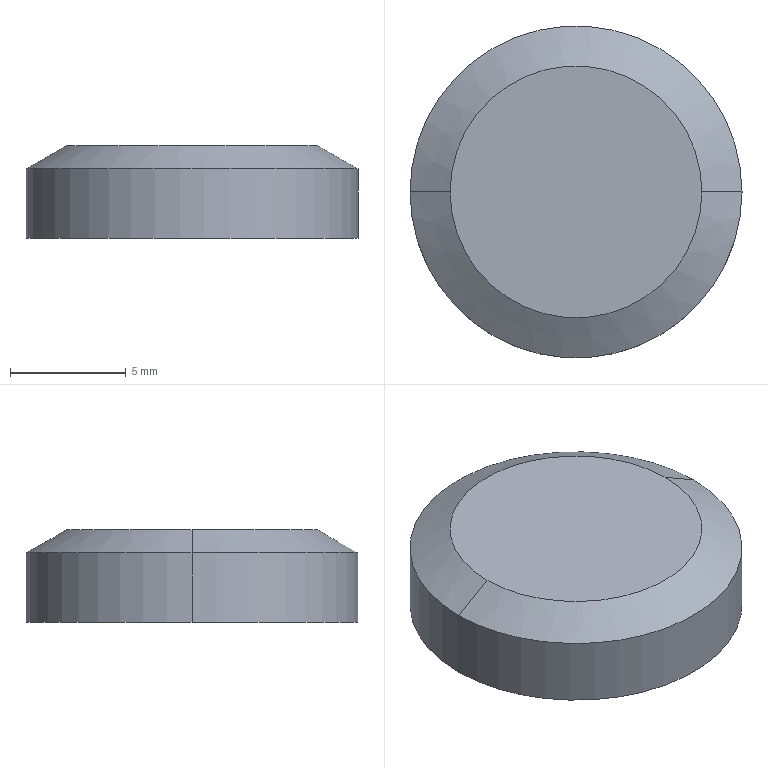CAM job | Mastercam | mm | 4 operations | part box 14.35 x 14.35 x 4
1. Contour (Ramp) | 6 - 6 平底刀
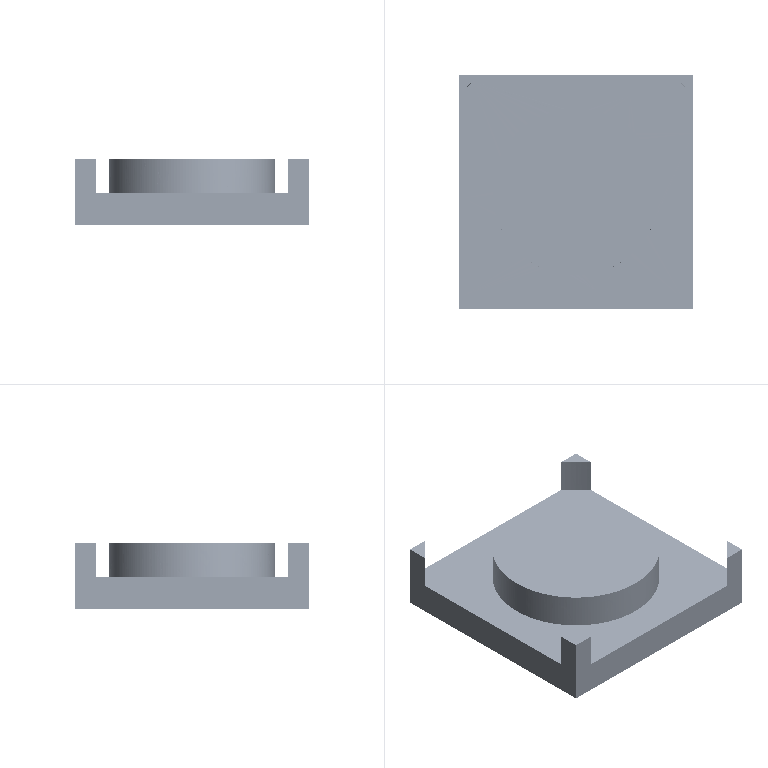2. Surface Finish Flowline | 6 - 6 平底刀
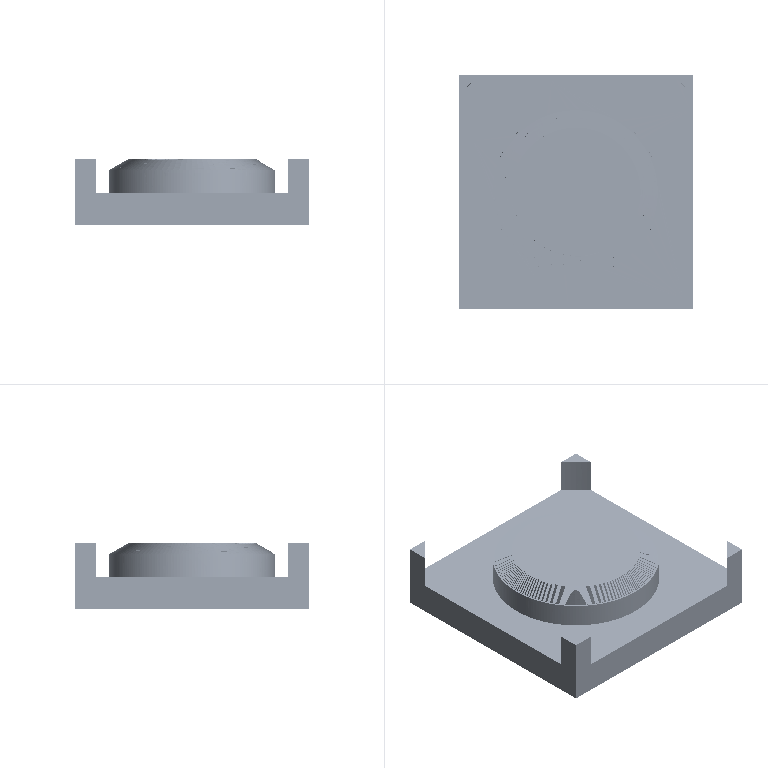3. Surface Finish Flowline | 22 - D6 -R1.0圆鼻铣刀
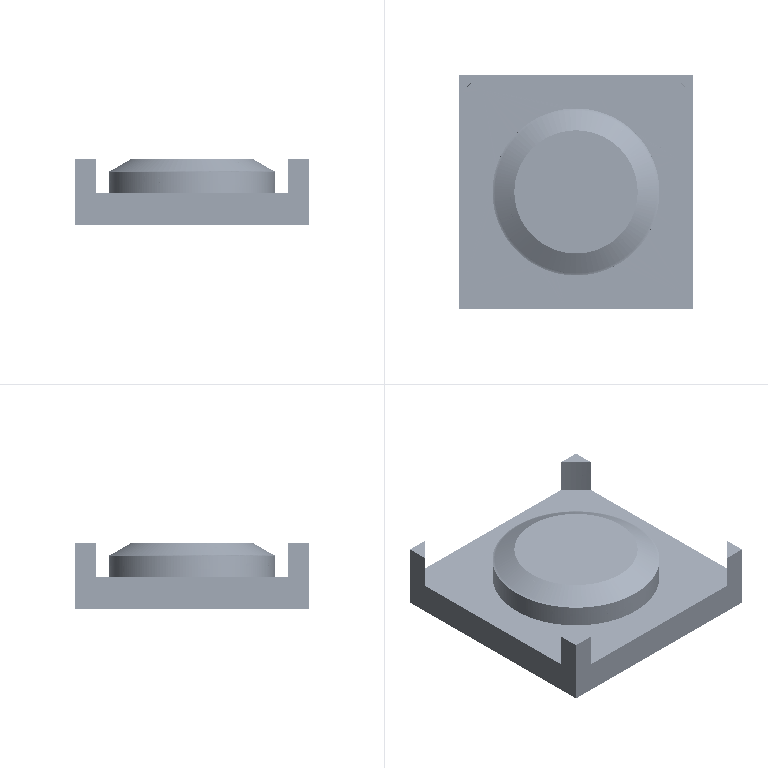4. Contour (2D) | 11 - 4 J平底刀